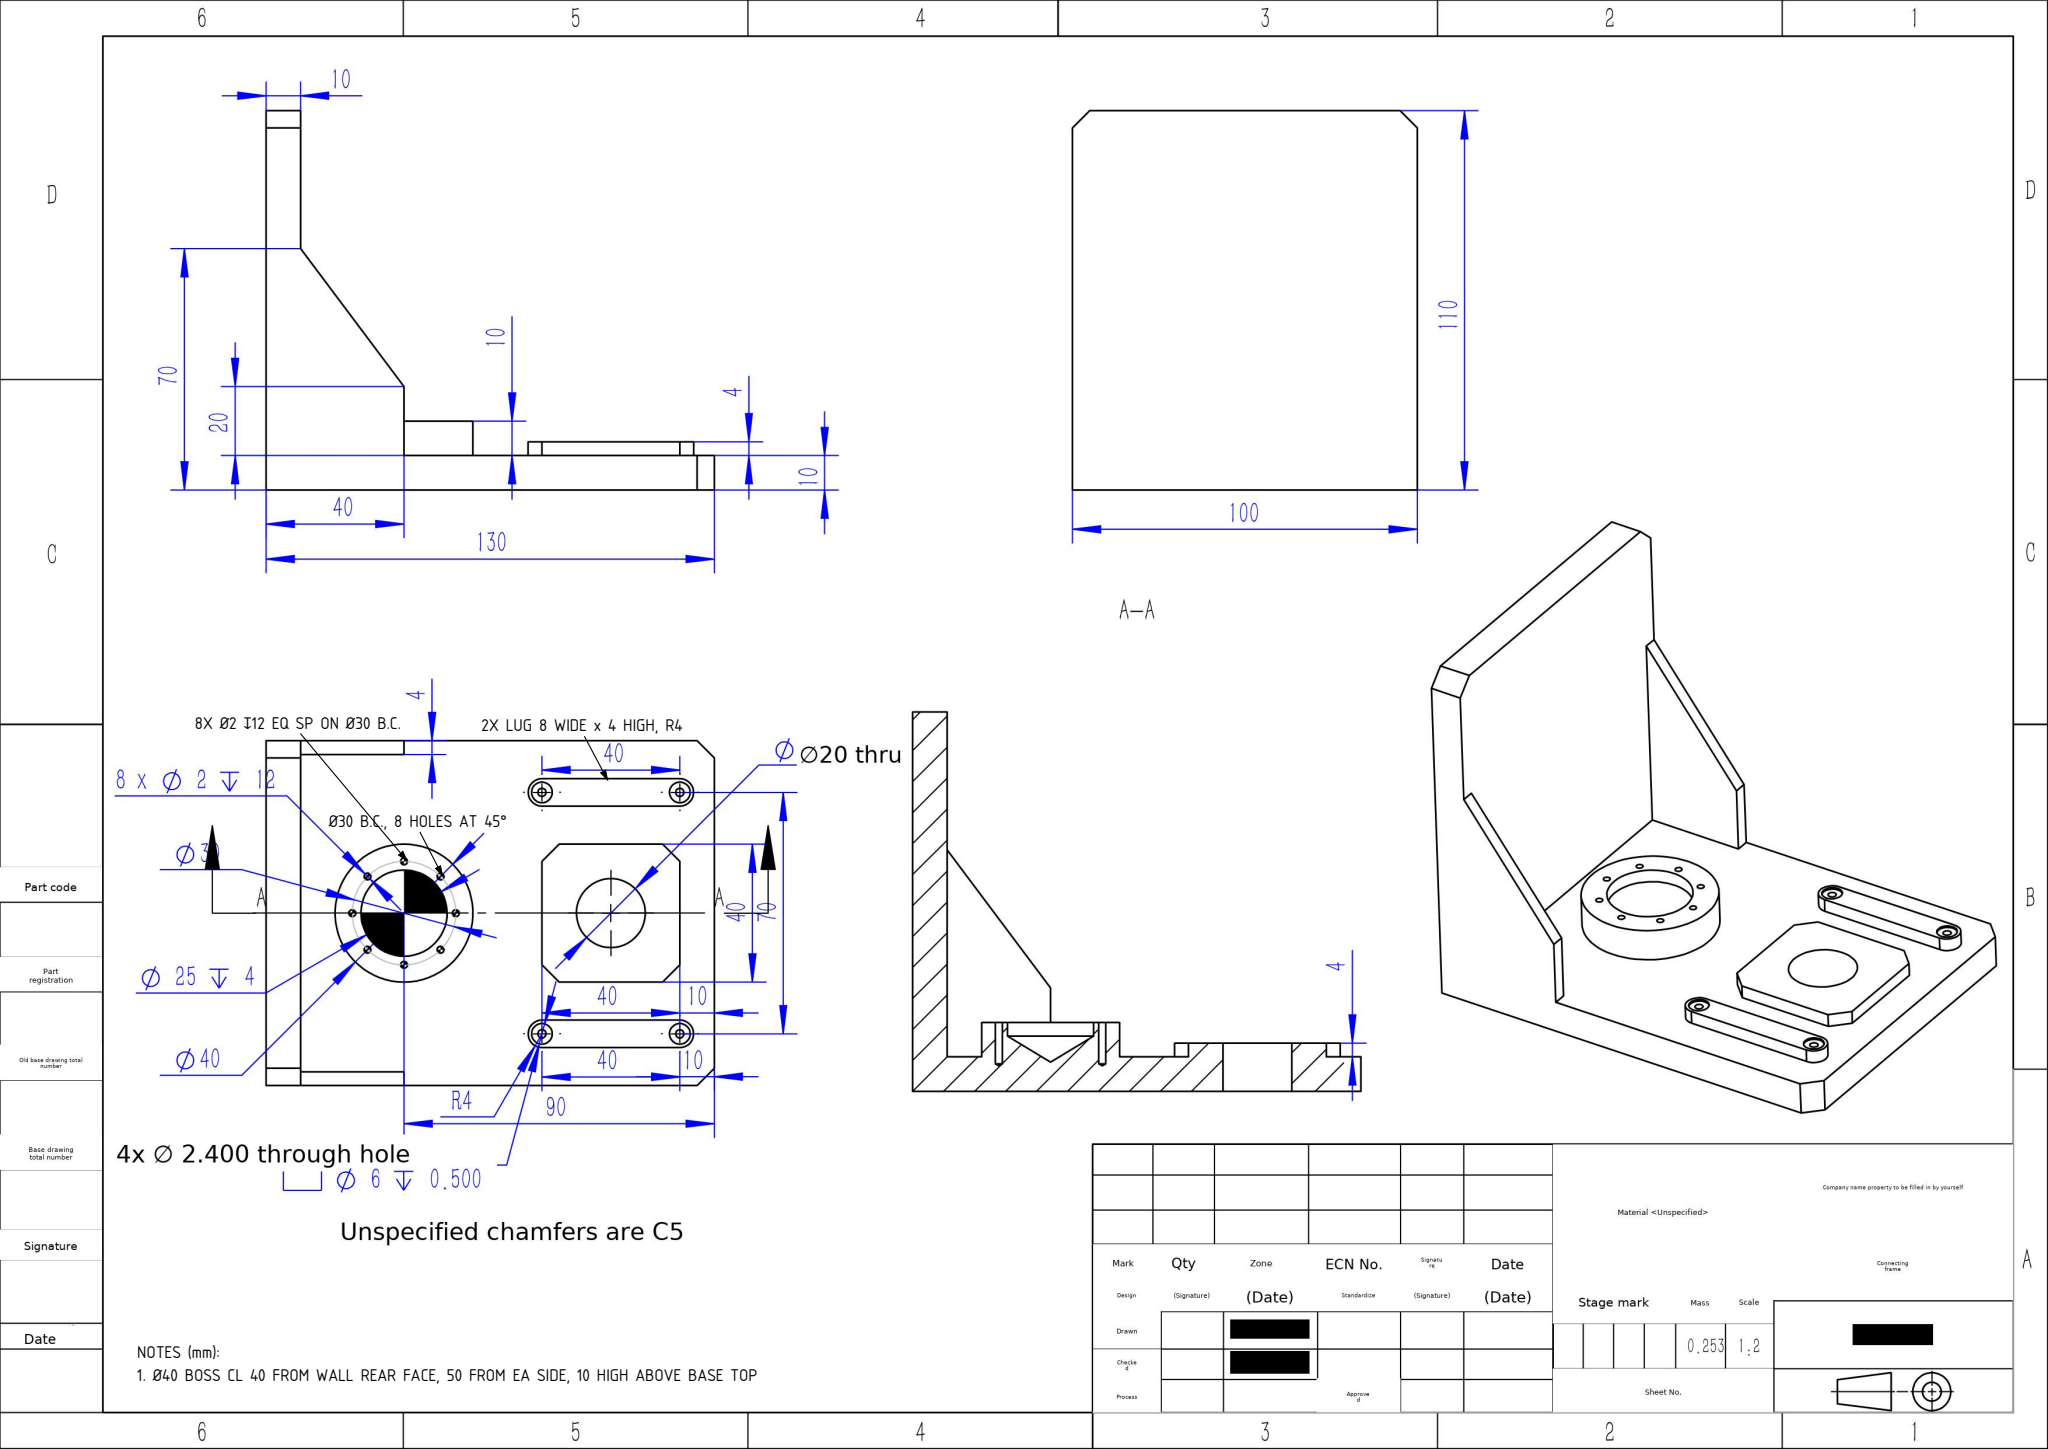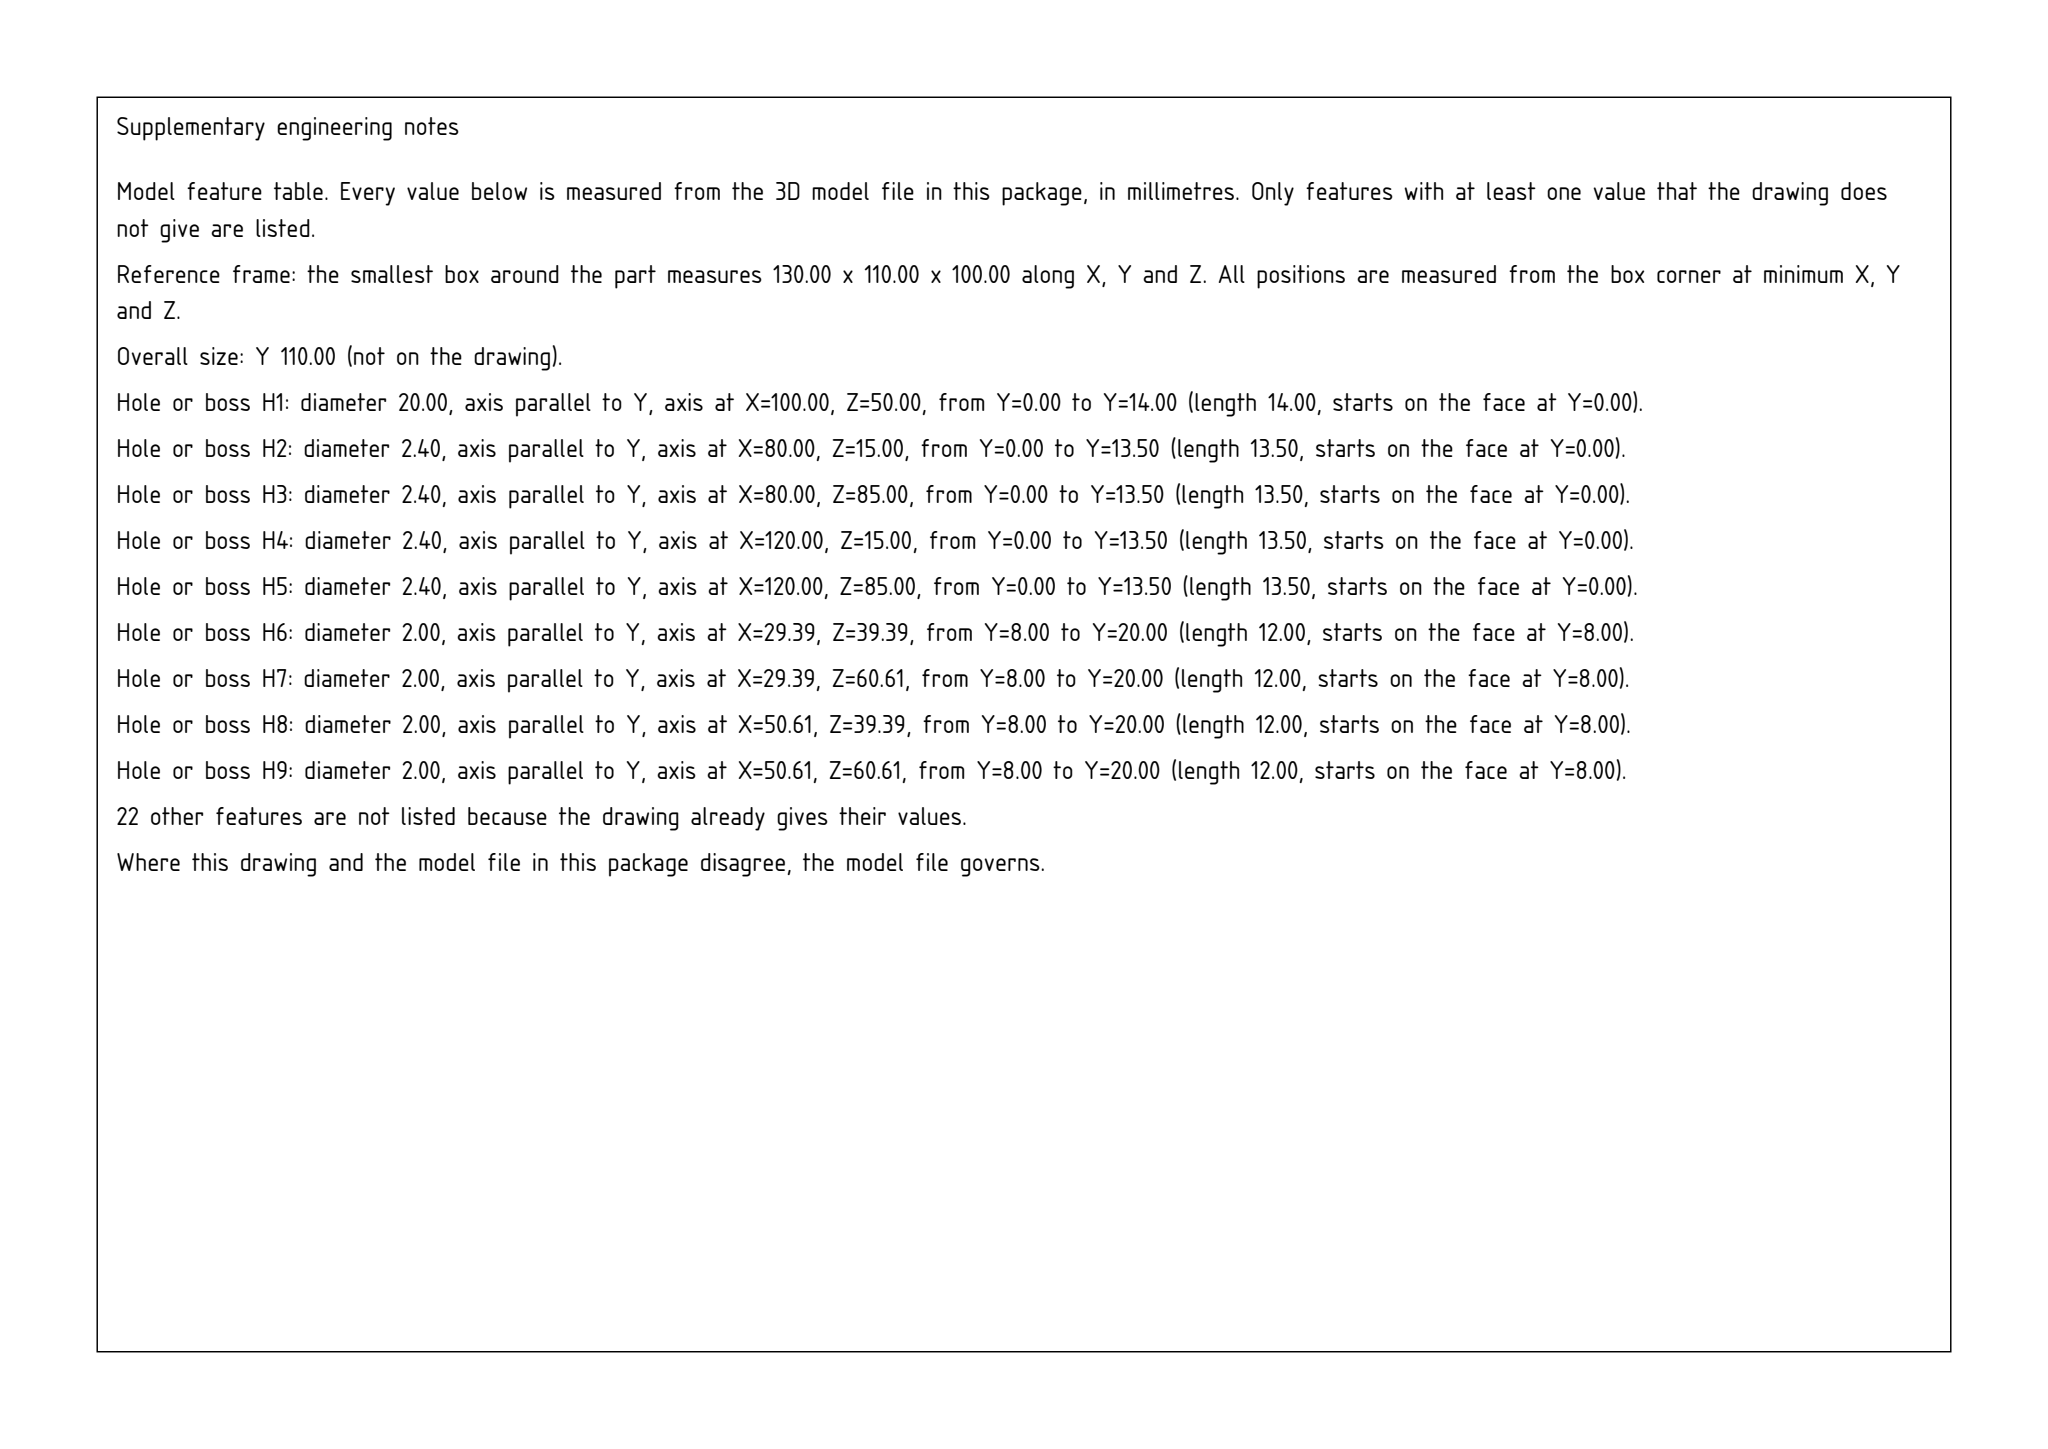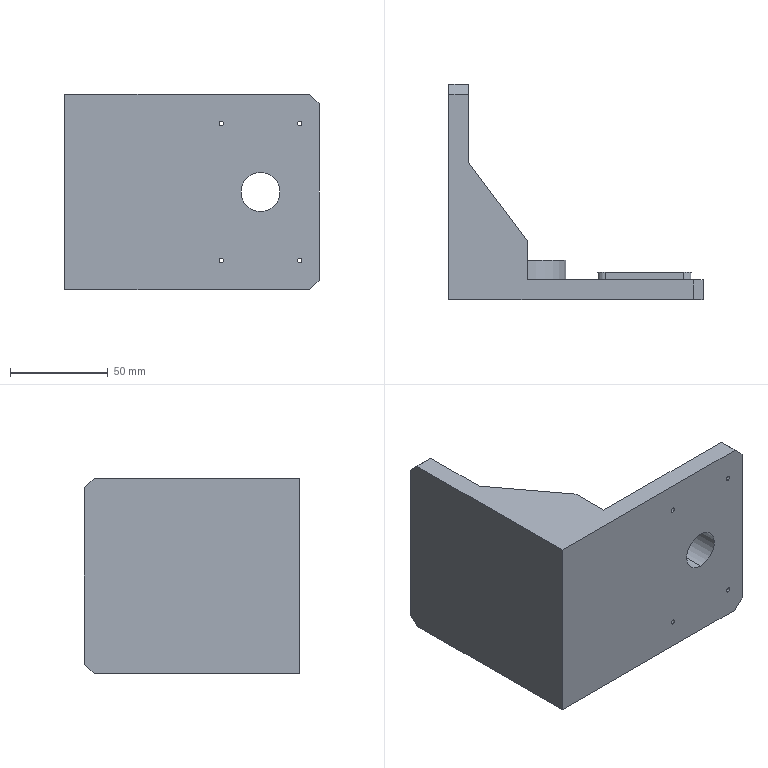Part | SolidWorks | mm | 1 solid | 98 faces | box 130 x 110 x 100 mm | volume 252630 mm3 | cylinder 42 | plane 38 | cone 18 | commonest cylinder face diameters 2 x16 6 x8 2.4 x8 8 x4 25 x2 40 x2 20 x2
Drawing notes:
Ø40 BOSS CL 40 FROM WALL REAR FACE, 50 FROM EA SIDE, 10 HIGH ABOVE BASE TOP | from the solid: Ø40 cyl at x=40, z=50, length 10 (y=10 to 20); base top y=10; bbox 130 x 100
2X LUG 8 WIDE X 4 HIGH, R4 ENDS, HOLE CL 40 APART, 15 FROM EA SIDE | from the solid: Ø8 cyls L4 (y=10 to 14) at (80,15),(120,15),(80,85),(120,85); Ø2.4 THRU + Ø6 DP 0.5
8X Ø2 DP 12 EQ SP ON Ø30 B.C., CTR'D ON Ø40 BOSS | from the solid: Eight Ø2.0 holes, axis y, at (25,50),(55,50),(40,35),(40,65),(29.4,39.4),(29.4,60.6),(50.6,39.4),(50.6,60.6) = R15 about boss axis (40,50); depth y 8->20 = 12
BOLT CIRCLE FOR 8X Ø2 HOLES = Ø30 (45° SPACING) | from the solid: Hole centers lie 15.0 from Ø40 boss axis (40,50); 8 holes at 45° increments
build123d program:
from build123d import *

# Parameters (mm, degrees)
EXTRUDE_THIN1_DEPTH                       = 50
SKETCH2_W                                 = 40
SKETCH2_H                                 = 40
BOSS_EXTRUDE1_DEPTH                       = 4
BOSS_EXTRUDE2_DEPTH                       = 4
SKETCH4_R                                 = 10
CUT_EXTRUDE1_DEPTH                        = 162.604
CHAMFER1_SIZE                             = 5
SKETCH5_R                                 = 20
BOSS_EXTRUDE3_DEPTH                       = 10
F_2_0MM_DOWEL_PIN_HOLE1_D                 = 2
F_2_0MM_DOWEL_PIN_HOLE1_DEPTH             = 12
F_2_0MM_DOWEL_PIN_HOLE1_TIP               = 0.6009
F_25_0MM_DOWEL_PIN_HOLE1_D                = 25
F_25_0MM_DOWEL_PIN_HOLE1_DEPTH            = 4
F_25_0MM_DOWEL_PIN_HOLE1_TIP              = 7.511
M2_HEX_HEAD_BOLT_COUNTERBORE1_D           = 2.4
M2_HEX_HEAD_BOLT_COUNTERBORE1_CBORE_D     = 6
M2_HEX_HEAD_BOLT_COUNTERBORE1_CBORE_DEPTH = 0.5


with BuildPart() as part:
    # Sketch1 → Extrude-Thin1 (new, symmetric)
    with BuildSketch(Plane.XY):
        Polygon((0, 100), (0, 0), (120, 0), (120, -10), (-10, -10), (-10, 100), align=None)
    extrude(amount=EXTRUDE_THIN1_DEPTH, both=True)

    # Sketch2 → Boss-Extrude1 (add)
    with BuildSketch(Plane(origin=(0, 0, 0), x_dir=(1, 0, 0), z_dir=(0, 1, 0))):
        with Locations((90, 0)):
            Rectangle(SKETCH2_W, SKETCH2_H)
        with BuildLine():
            Line((70, 39), (110, 39))
            ThreePointArc((110, 39), (114, 35), (110, 31))
            Line((110, 31), (70, 31))
            ThreePointArc((70, 31), (66, 35), (70, 39))
        make_face()
        with BuildLine():
            Line((70, -31), (110, -31))
            ThreePointArc((110, -31), (114, -35), (110, -39))
            Line((110, -39), (70, -39))
            ThreePointArc((70, -39), (66, -35), (70, -31))
        make_face()
    extrude(amount=BOSS_EXTRUDE1_DEPTH)

    # Sketch3 → Boss-Extrude2 (add)
    with BuildSketch(Plane.XY.offset(50)):
        Polygon((0, 60), (30, 20), (30, 0), (0, 0), align=None)
    boss_extrude2 = extrude(amount=-BOSS_EXTRUDE2_DEPTH)

    # Mirror2: Boss-Extrude2 across plane
    add(boss_extrude2.mirror(Plane.XY))

    # Sketch4 → Cut-Extrude1 (cut, through all)
    with BuildSketch(Plane(origin=(0, 4, 0), x_dir=(1, 0, 0), z_dir=(0, 1, 0))):
        with Locations(Location((90, 0, 0), (0, 0, 270))):
            Circle(SKETCH4_R)
    extrude(amount=-CUT_EXTRUDE1_DEPTH, mode=Mode.SUBTRACT)

    # Chamfer1
    chamfer1_edges = [part.edges().sort_by_distance(p)[0] for p in [
        (-5, 100, 50),
        (70, 2, -20),
        (70, 2, 20),
        (110, 2, 20),
        (110, 2, -20),
        (-5, 100, -50),
        (120, -5, -50),
        (120, -5, 50),
    ]]
    chamfer(chamfer1_edges, length=CHAMFER1_SIZE)

    # Sketch5 → Boss-Extrude3 (add)
    with BuildSketch(Plane(origin=(0, 0, 0), x_dir=(1, 0, 0), z_dir=(0, 1, 0))):
        with Locations(Location((30, 0, 0), (0, 0, 270))):
            Circle(SKETCH5_R)
    extrude(amount=BOSS_EXTRUDE3_DEPTH)

    # 2.0mm Dowel Pin Hole1
    with Locations(Plane(origin=(0, 10, 0), x_dir=(1, 0, 0), z_dir=(0, 1, 0))):
        with Locations((19.393, 10.607), (30, 15), (40.607, 10.607), (45, 0), (40.607, -10.607), (30, -15), (19.393, -10.607), (15, 0)):
            Hole(F_2_0MM_DOWEL_PIN_HOLE1_D / 2, depth=F_2_0MM_DOWEL_PIN_HOLE1_DEPTH)
            with Locations((0, 0, -(F_2_0MM_DOWEL_PIN_HOLE1_DEPTH + F_2_0MM_DOWEL_PIN_HOLE1_TIP / 2))):  # 118° drill point
                Cone(0, F_2_0MM_DOWEL_PIN_HOLE1_D / 2, F_2_0MM_DOWEL_PIN_HOLE1_TIP, mode=Mode.SUBTRACT)

    # 25.0mm Dowel Pin Hole1
    with Locations(Plane(origin=(0, 10, 0), x_dir=(1, 0, 0), z_dir=(0, 1, 0))):
        with Locations((30, 0)):
            Hole(F_25_0MM_DOWEL_PIN_HOLE1_D / 2, depth=F_25_0MM_DOWEL_PIN_HOLE1_DEPTH)
            with Locations((0, 0, -(F_25_0MM_DOWEL_PIN_HOLE1_DEPTH + F_25_0MM_DOWEL_PIN_HOLE1_TIP / 2))):  # 118° drill point
                Cone(0, F_25_0MM_DOWEL_PIN_HOLE1_D / 2, F_25_0MM_DOWEL_PIN_HOLE1_TIP, mode=Mode.SUBTRACT)

    # M2 Hex Head Bolt Counterbore1 (through all)
    with Locations(Plane(origin=(0, 4, 0), x_dir=(1, 0, 0), z_dir=(0, 1, 0))):
        with Locations((70, -35), (110, -35), (110, 35), (70, 35)):
            CounterBoreHole(M2_HEX_HEAD_BOLT_COUNTERBORE1_D / 2, M2_HEX_HEAD_BOLT_COUNTERBORE1_CBORE_D / 2, M2_HEX_HEAD_BOLT_COUNTERBORE1_CBORE_DEPTH)


solid = part.part